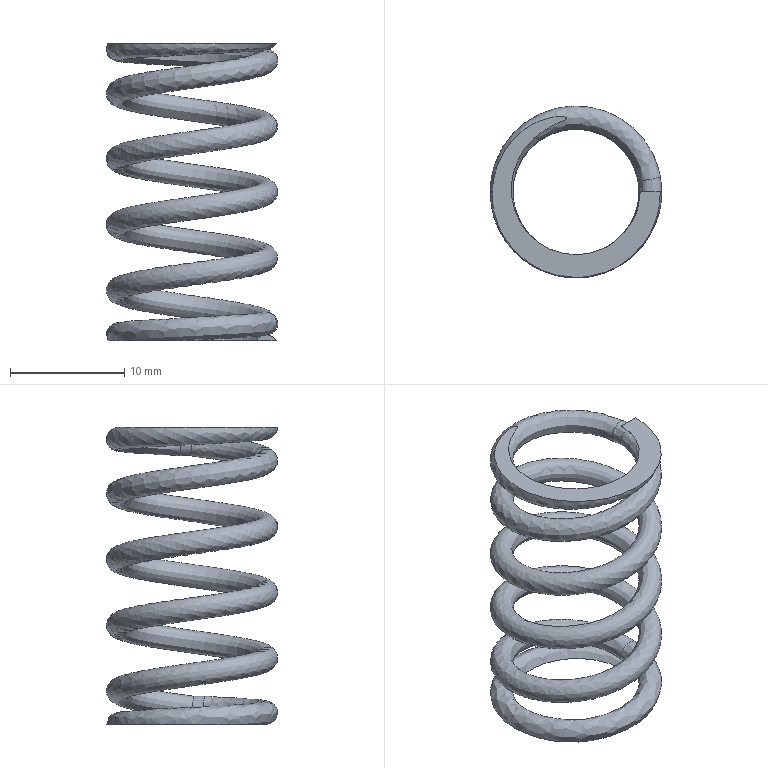Component | NX | SPRING_2 | 1 solid | 9 faces | volume 697 mm3 | spline 5 | plane 4